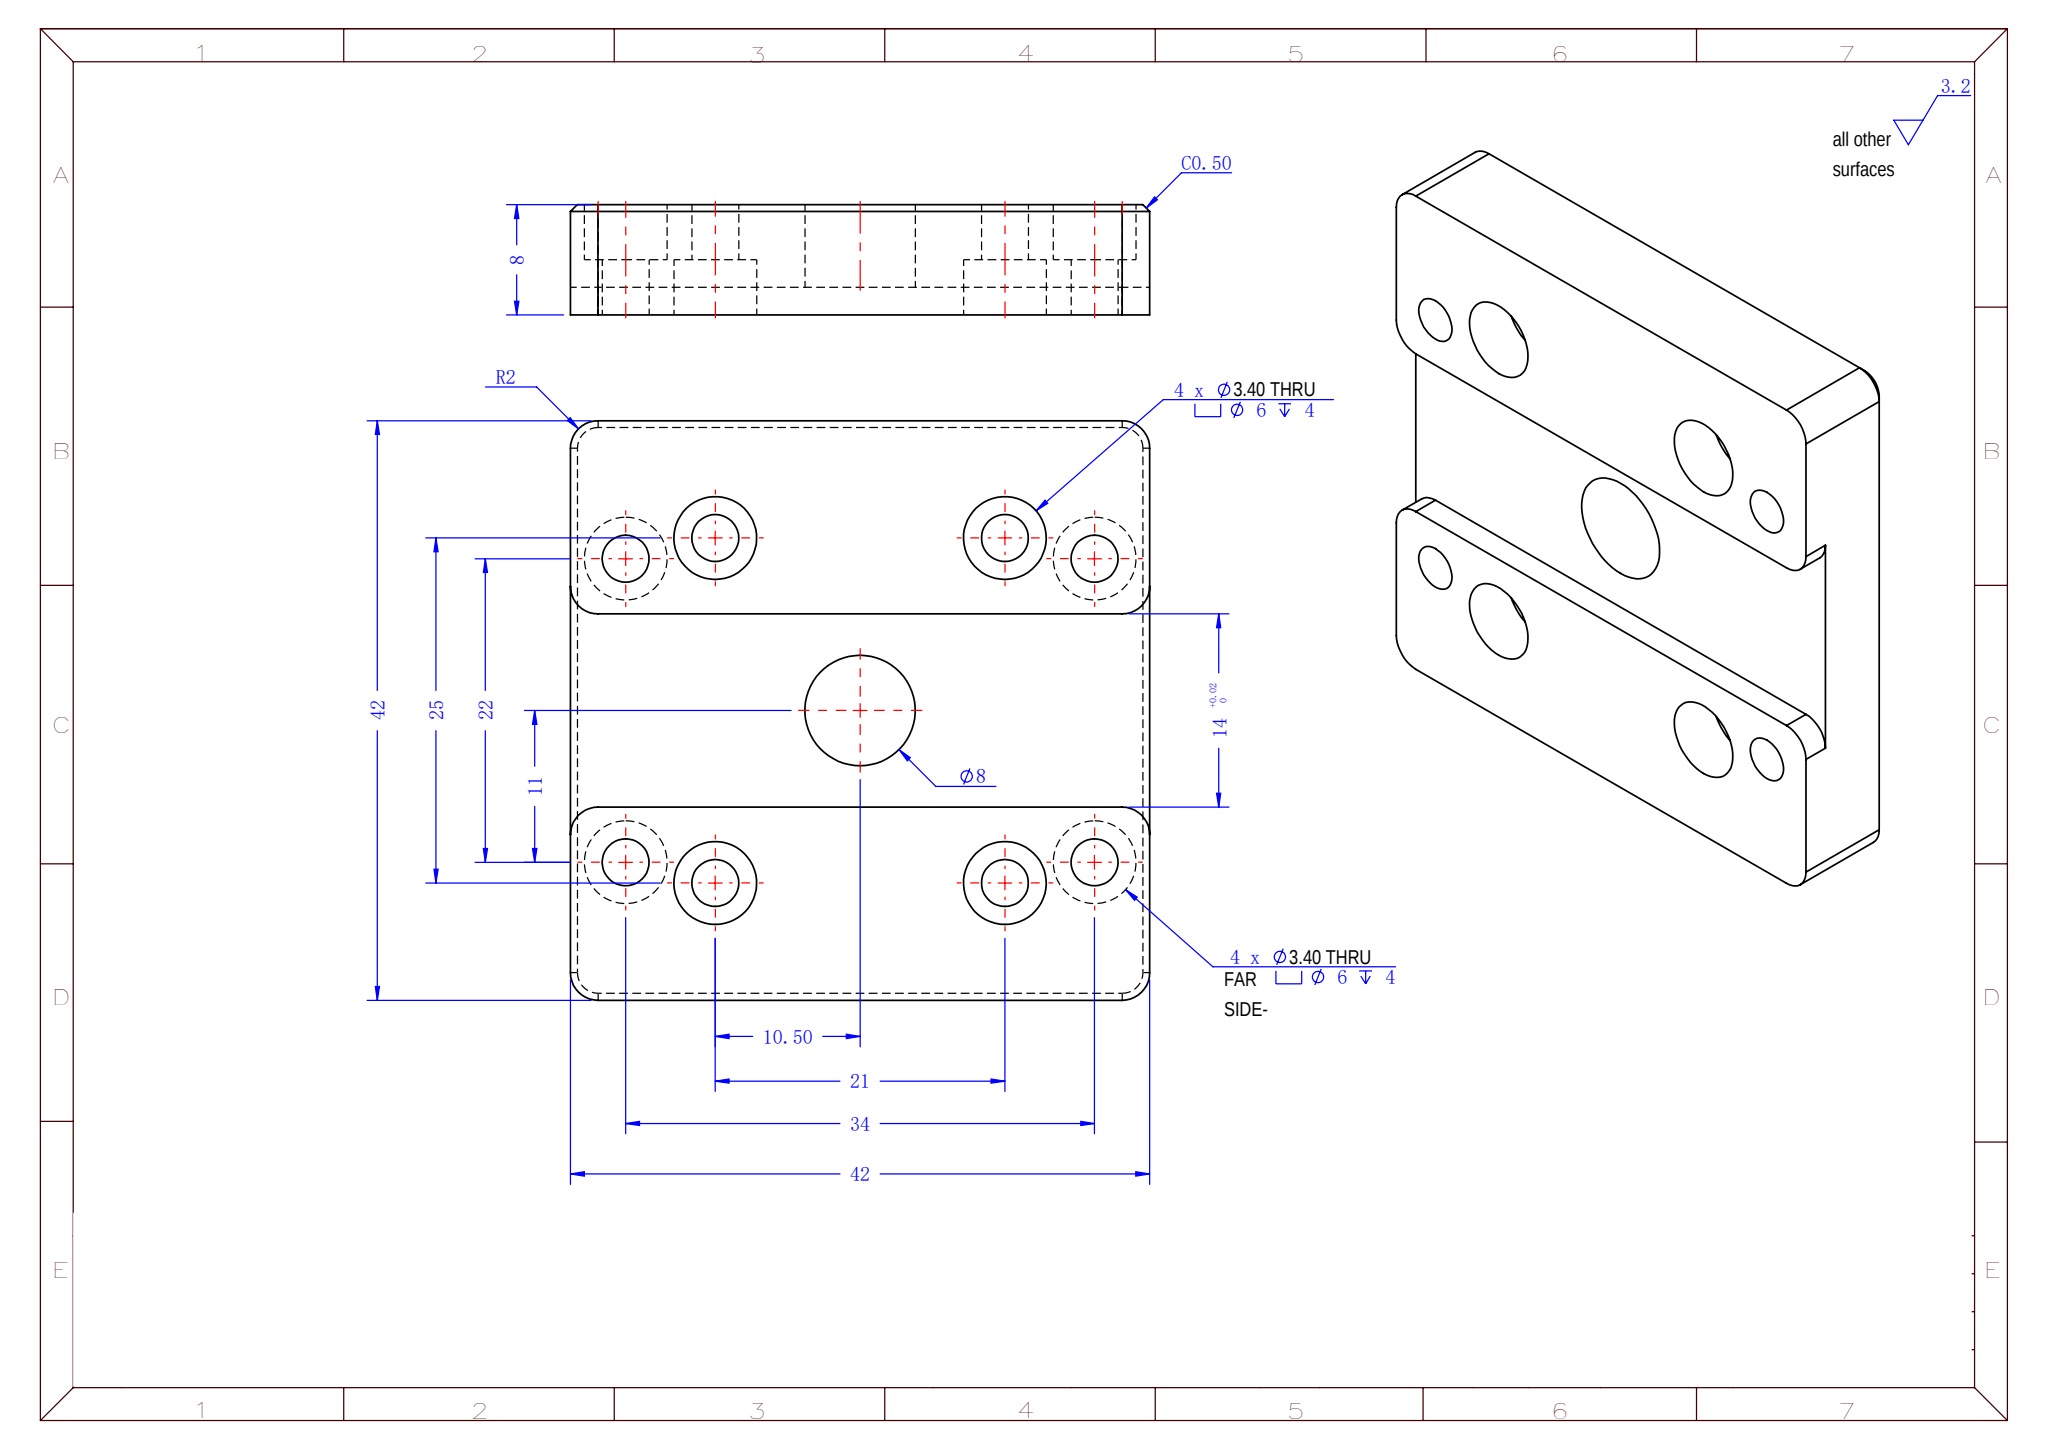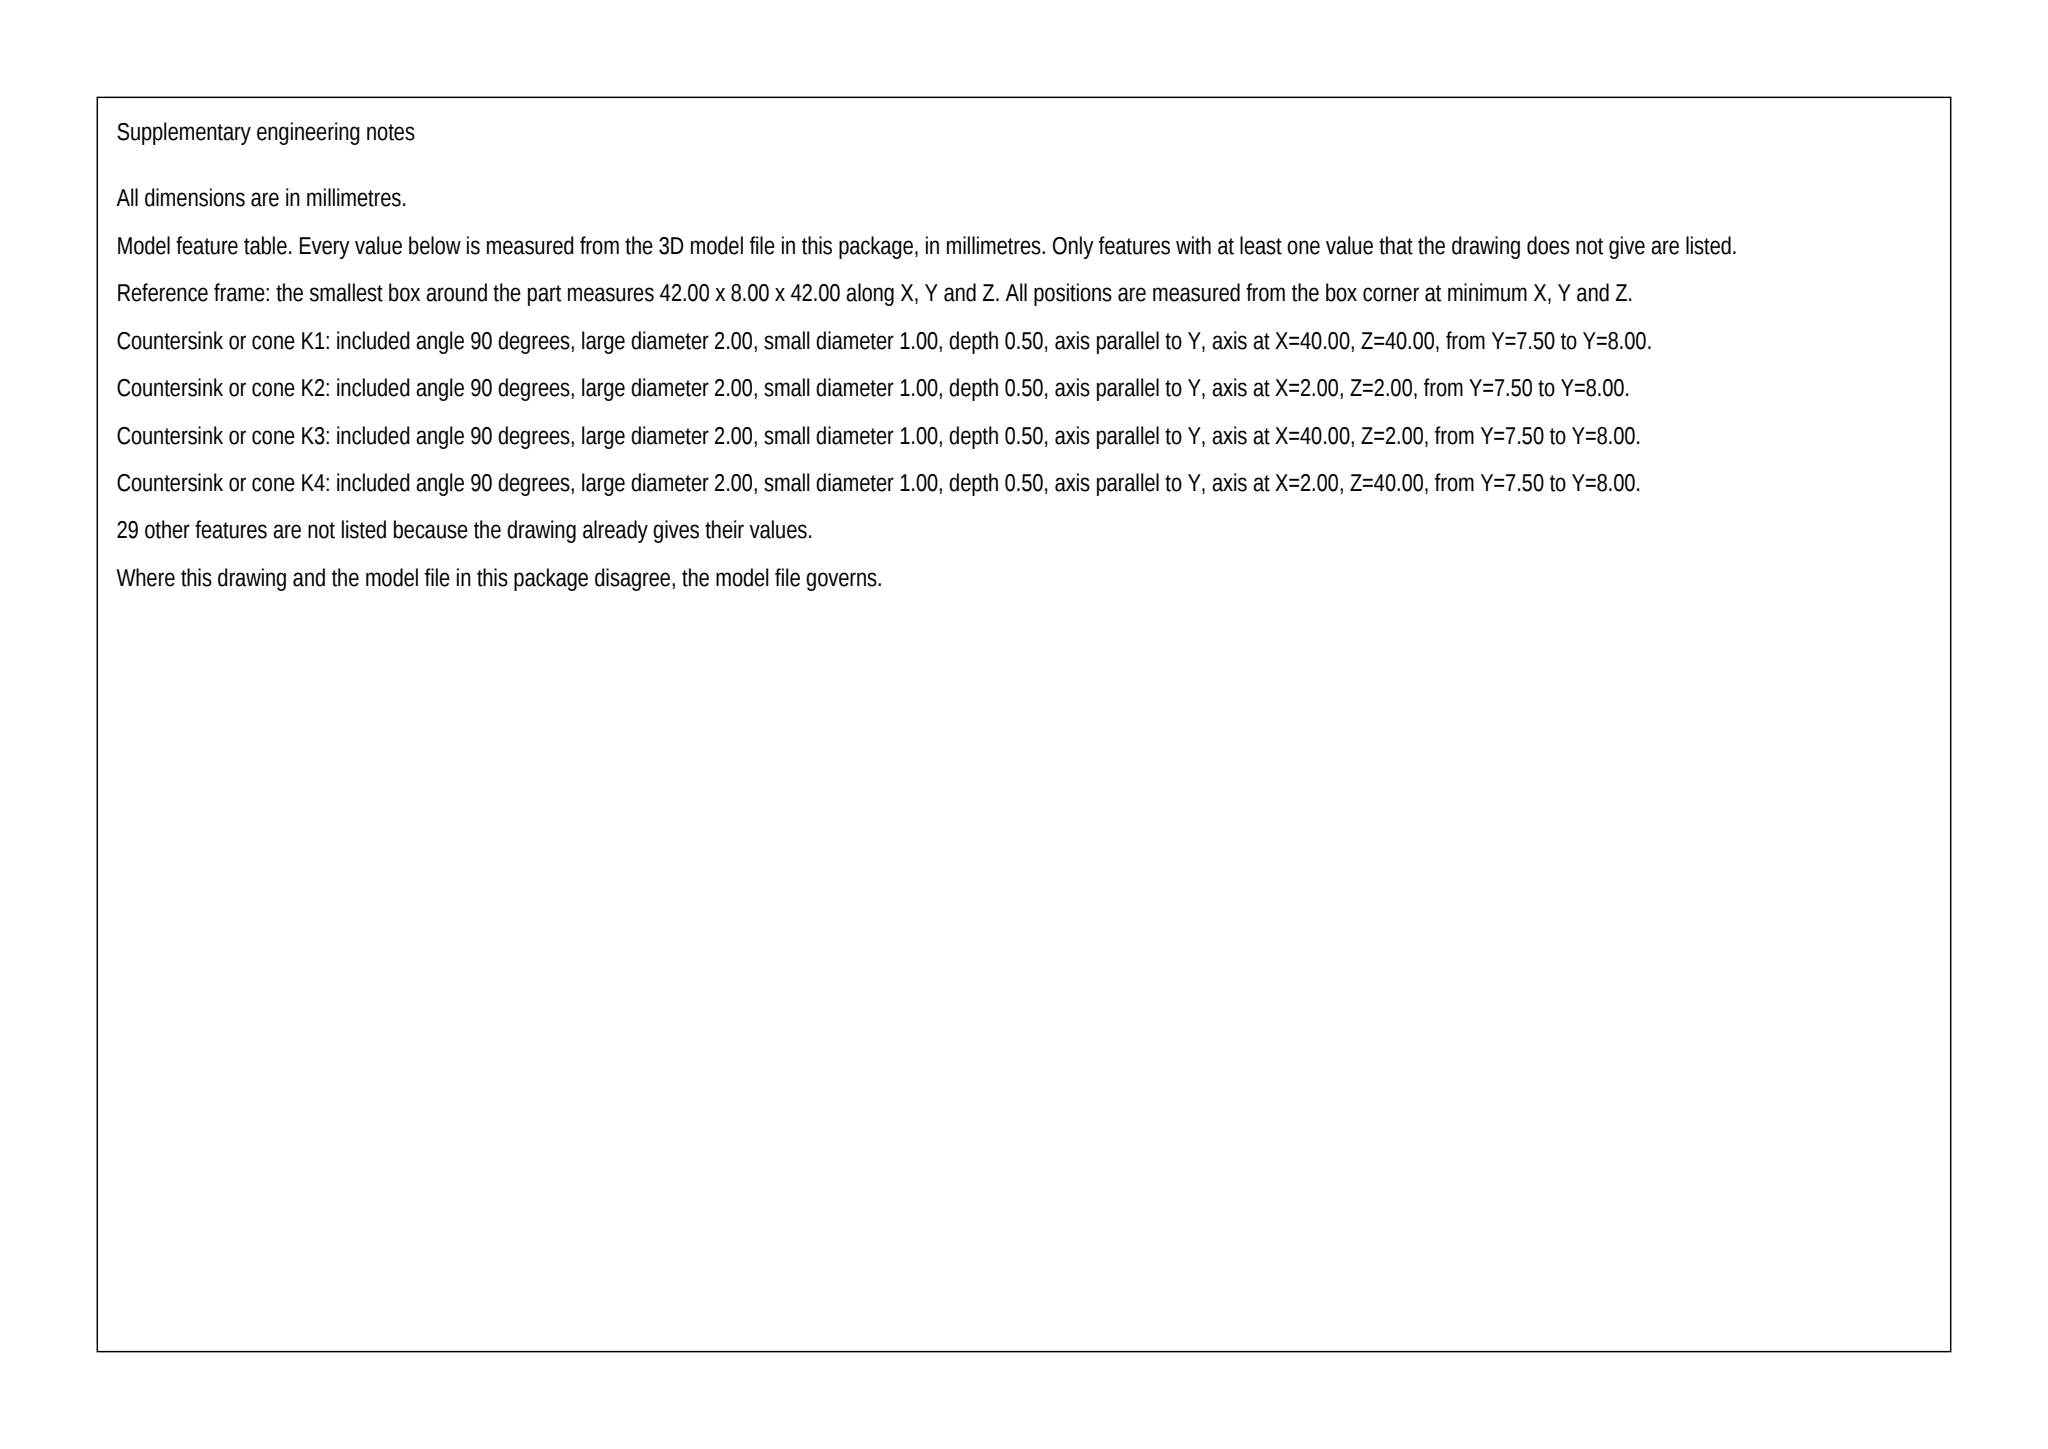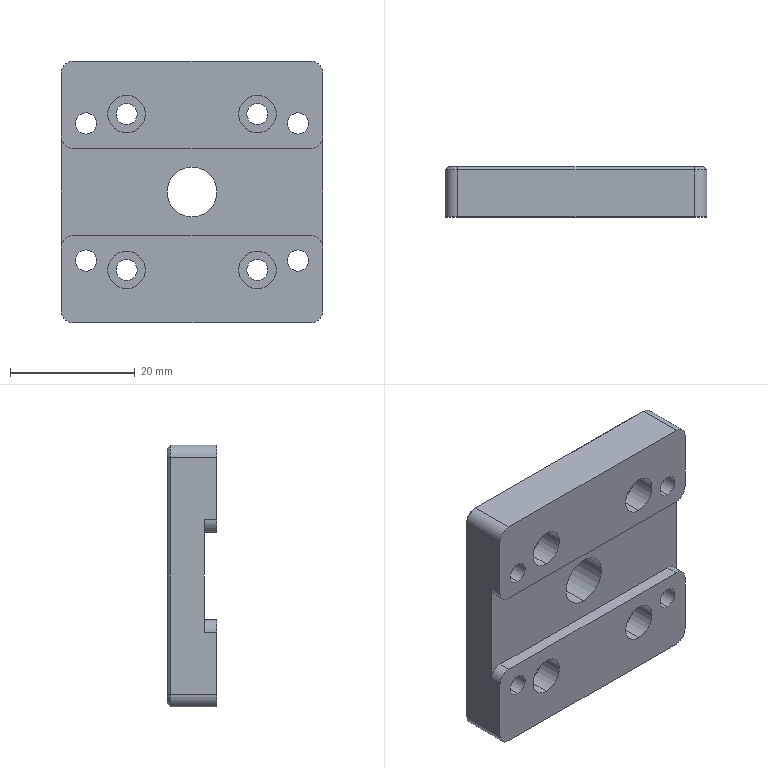Part | SolidWorks | mm | 1 solid | 68 faces | box 42 x 8 x 42 mm | volume 11384 mm3 | cylinder 42 | plane 22 | cone 4 | commonest cylinder face diameters 6 x16 3.4 x16 4 x8 8 x2
build123d program:
from build123d import *

# Parameters (mm, degrees)
SKETCH1_W                                           = 42
SKETCH1_H                                           = 42
BOSS_EXTRUDE1_DEPTH                                 = 4
CYLINDRICAL_COUNTERSUNK_HOLE_FOR_M3_HEX_D           = 3.4
CYLINDRICAL_COUNTERSUNK_HOLE_FOR_M3_HEX_CBORE_D     = 6
CYLINDRICAL_COUNTERSUNK_HOLE_FOR_M3_HEX_CBORE_DEPTH = 4
SKETCH3_W                                           = 42
SKETCH3_H                                           = 14
CUT_EXTRUDE5_DEPTH                                  = 2
FILLET3_R                                           = 2
CYLINDRICAL_COUNTERSUNK_HOLE_FOR_M3_2_D             = 3.4
CYLINDRICAL_COUNTERSUNK_HOLE_FOR_M3_2_CBORE_D       = 6
CYLINDRICAL_COUNTERSUNK_HOLE_FOR_M3_2_CBORE_DEPTH   = 4
CHAMFER3_SIZE                                       = 0.5
SKETCH10_R                                          = 4
CUT_EXTRUDE6_DEPTH                                  = 31.757


with BuildPart() as part:
    # Sketch1 → Boss-Extrude1 (new, symmetric)
    with BuildSketch(Plane(origin=(0, 0, 0), x_dir=(1, 0, 0), z_dir=(0, 1, 0))):
        Rectangle(SKETCH1_W, SKETCH1_H)
    extrude(amount=BOSS_EXTRUDE1_DEPTH, both=True)

    # Cylindrical Countersunk Hole for M3 Hex (through all)
    with Locations(Plane.XZ.offset(4)):
        with Locations((-10.5, -12.5), (10.5, -12.5), (-10.5, 12.5), (10.5, 12.5)):
            CounterBoreHole(CYLINDRICAL_COUNTERSUNK_HOLE_FOR_M3_HEX_D / 2, CYLINDRICAL_COUNTERSUNK_HOLE_FOR_M3_HEX_CBORE_D / 2, CYLINDRICAL_COUNTERSUNK_HOLE_FOR_M3_HEX_CBORE_DEPTH)

    # Sketch3 → Cut-Extrude5 (cut)
    with BuildSketch(Plane.XZ.offset(4)):
        Rectangle(SKETCH3_W, SKETCH3_H)
    extrude(amount=-CUT_EXTRUDE5_DEPTH, mode=Mode.SUBTRACT)

    # Fillet3
    fillet3_edges = [part.edges().sort_by_distance(p)[0] for p in [
        (21, -3, 7),
        (21, -3, -7),
        (-21, -3, -7),
        (-21, -3, 7),
        (21, 0, 21),
        (-21, 0, 21),
        (-21, 0, -21),
        (21, 0, -21),
    ]]
    fillet(fillet3_edges, radius=FILLET3_R)

    # Cylindrical Countersunk Hole for M3  2 (through all)
    with Locations(Plane(origin=(0, 4, 0), x_dir=(1, 0, 0), z_dir=(0, 1, 0))):
        with Locations((-17, -11), (17, -11), (-17, 11), (17, 11)):
            CounterBoreHole(CYLINDRICAL_COUNTERSUNK_HOLE_FOR_M3_2_D / 2, CYLINDRICAL_COUNTERSUNK_HOLE_FOR_M3_2_CBORE_D / 2, CYLINDRICAL_COUNTERSUNK_HOLE_FOR_M3_2_CBORE_DEPTH)

    # Chamfer3
    chamfer3_edges = [part.edges().sort_by_distance(p)[0] for p in [
        (21, 4, 0),
        (0, 4, 21),
        (0, 4, -21),
        (-21, 4, 0),
        (-20.414, 4, -20.414),
        (20.414, 4, -20.414),
        (-20.414, 4, 20.414),
        (20.414, 4, 20.414),
    ]]
    chamfer(chamfer3_edges, length=CHAMFER3_SIZE)

    # Sketch10 → Cut-Extrude6 (cut, through all)
    with BuildSketch(Plane.XZ.offset(4)):
        with Locations(Location((0, 0, 0), (0, 0, 270))):
            Circle(SKETCH10_R)
    extrude(amount=-CUT_EXTRUDE6_DEPTH, mode=Mode.SUBTRACT)


solid = part.part